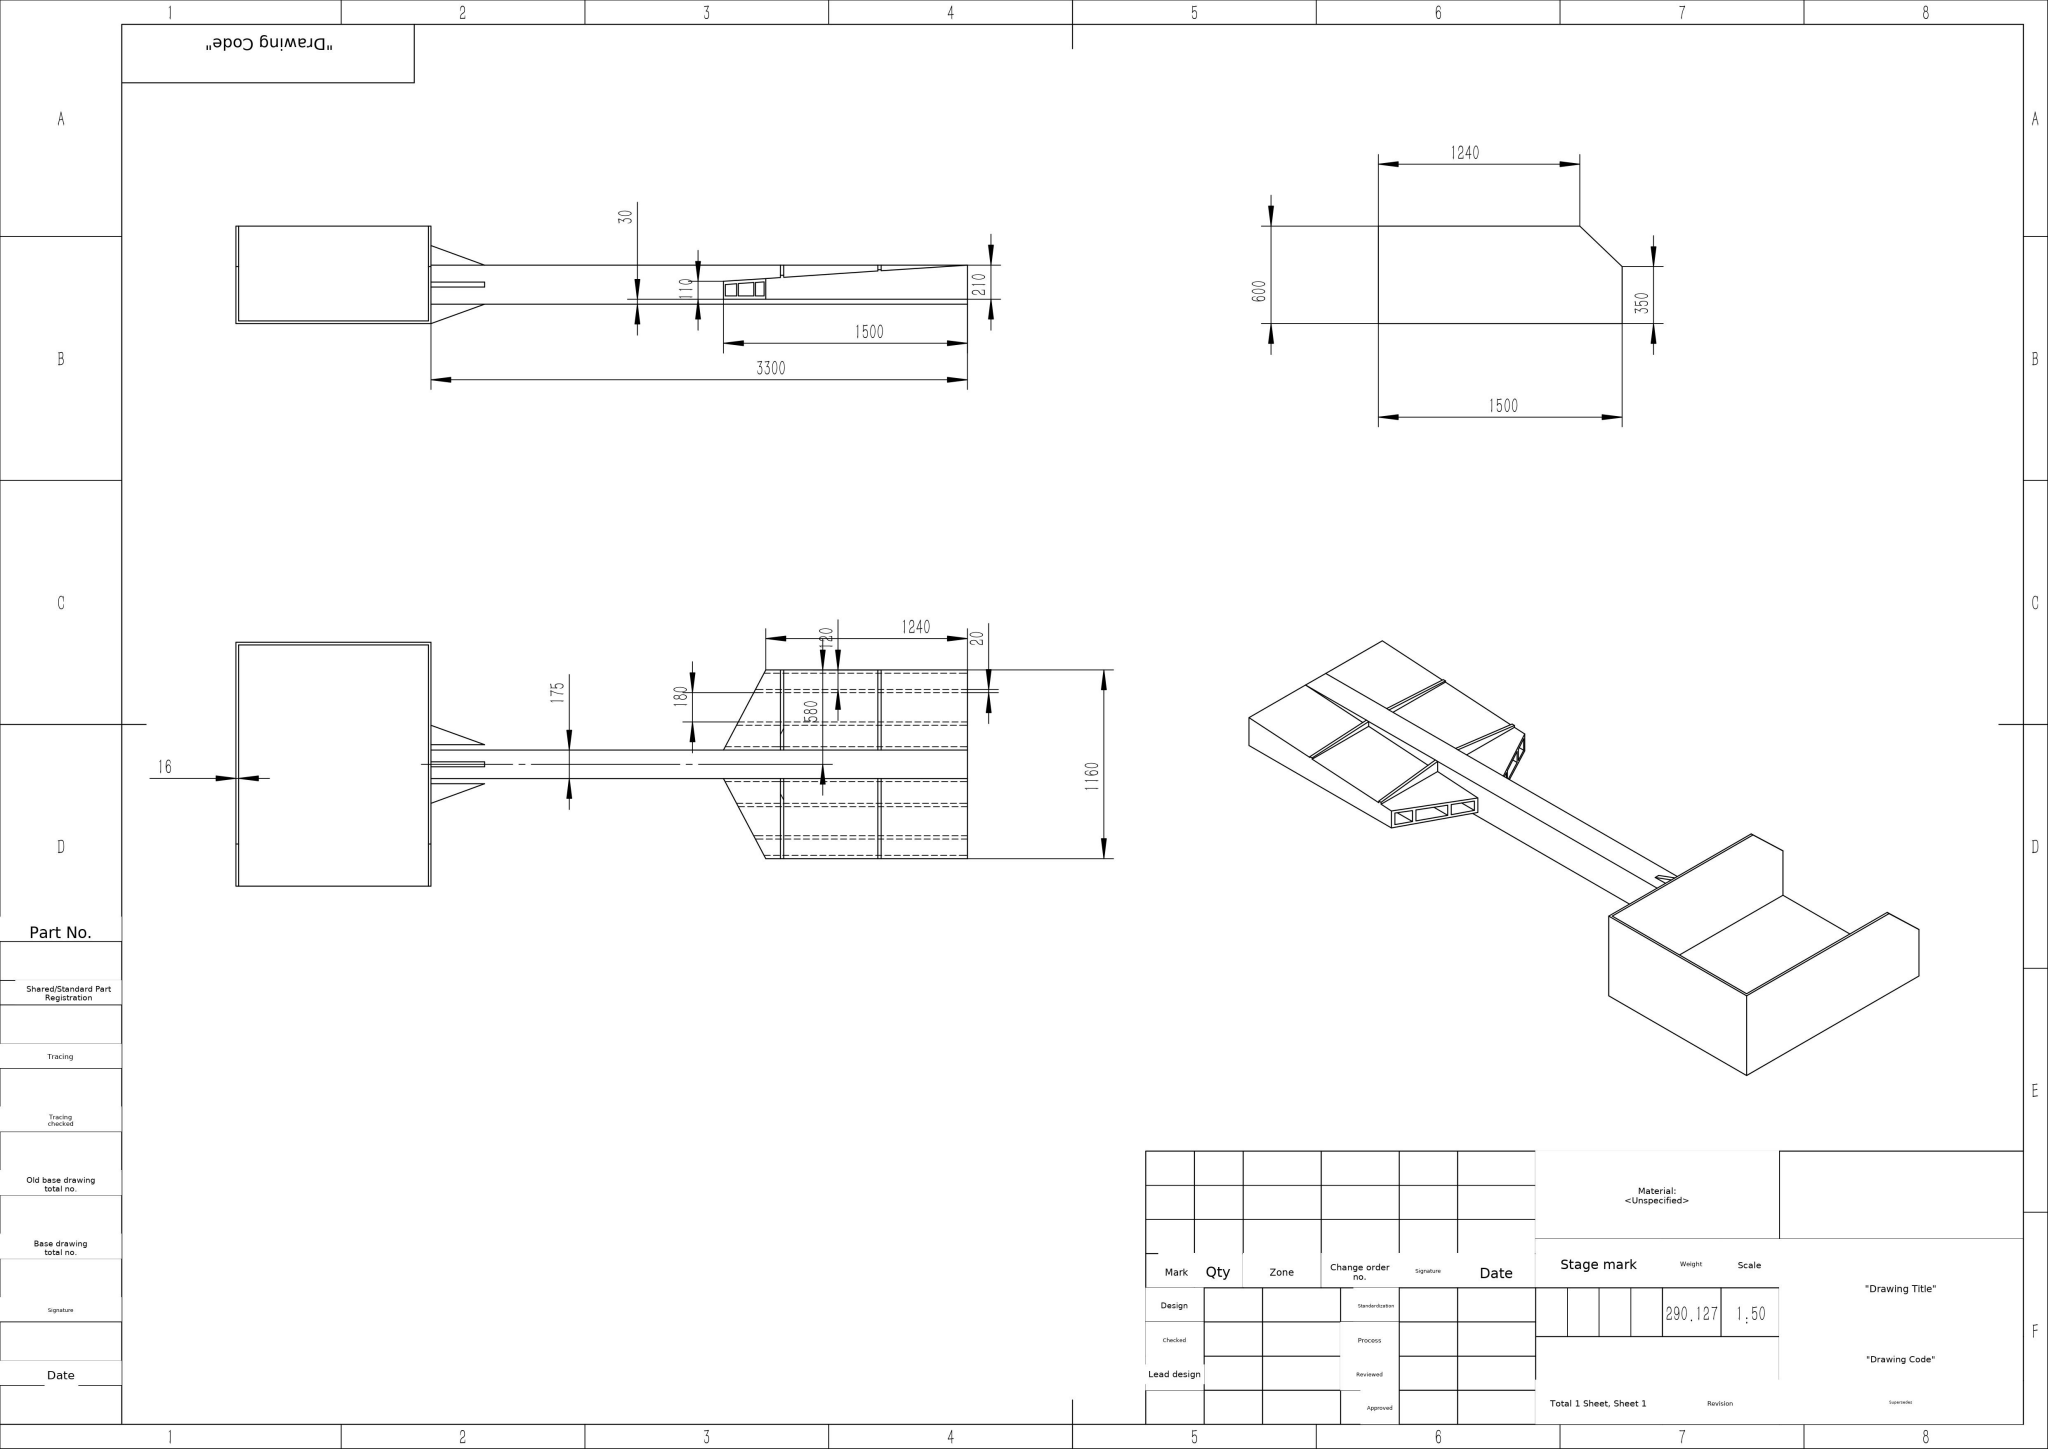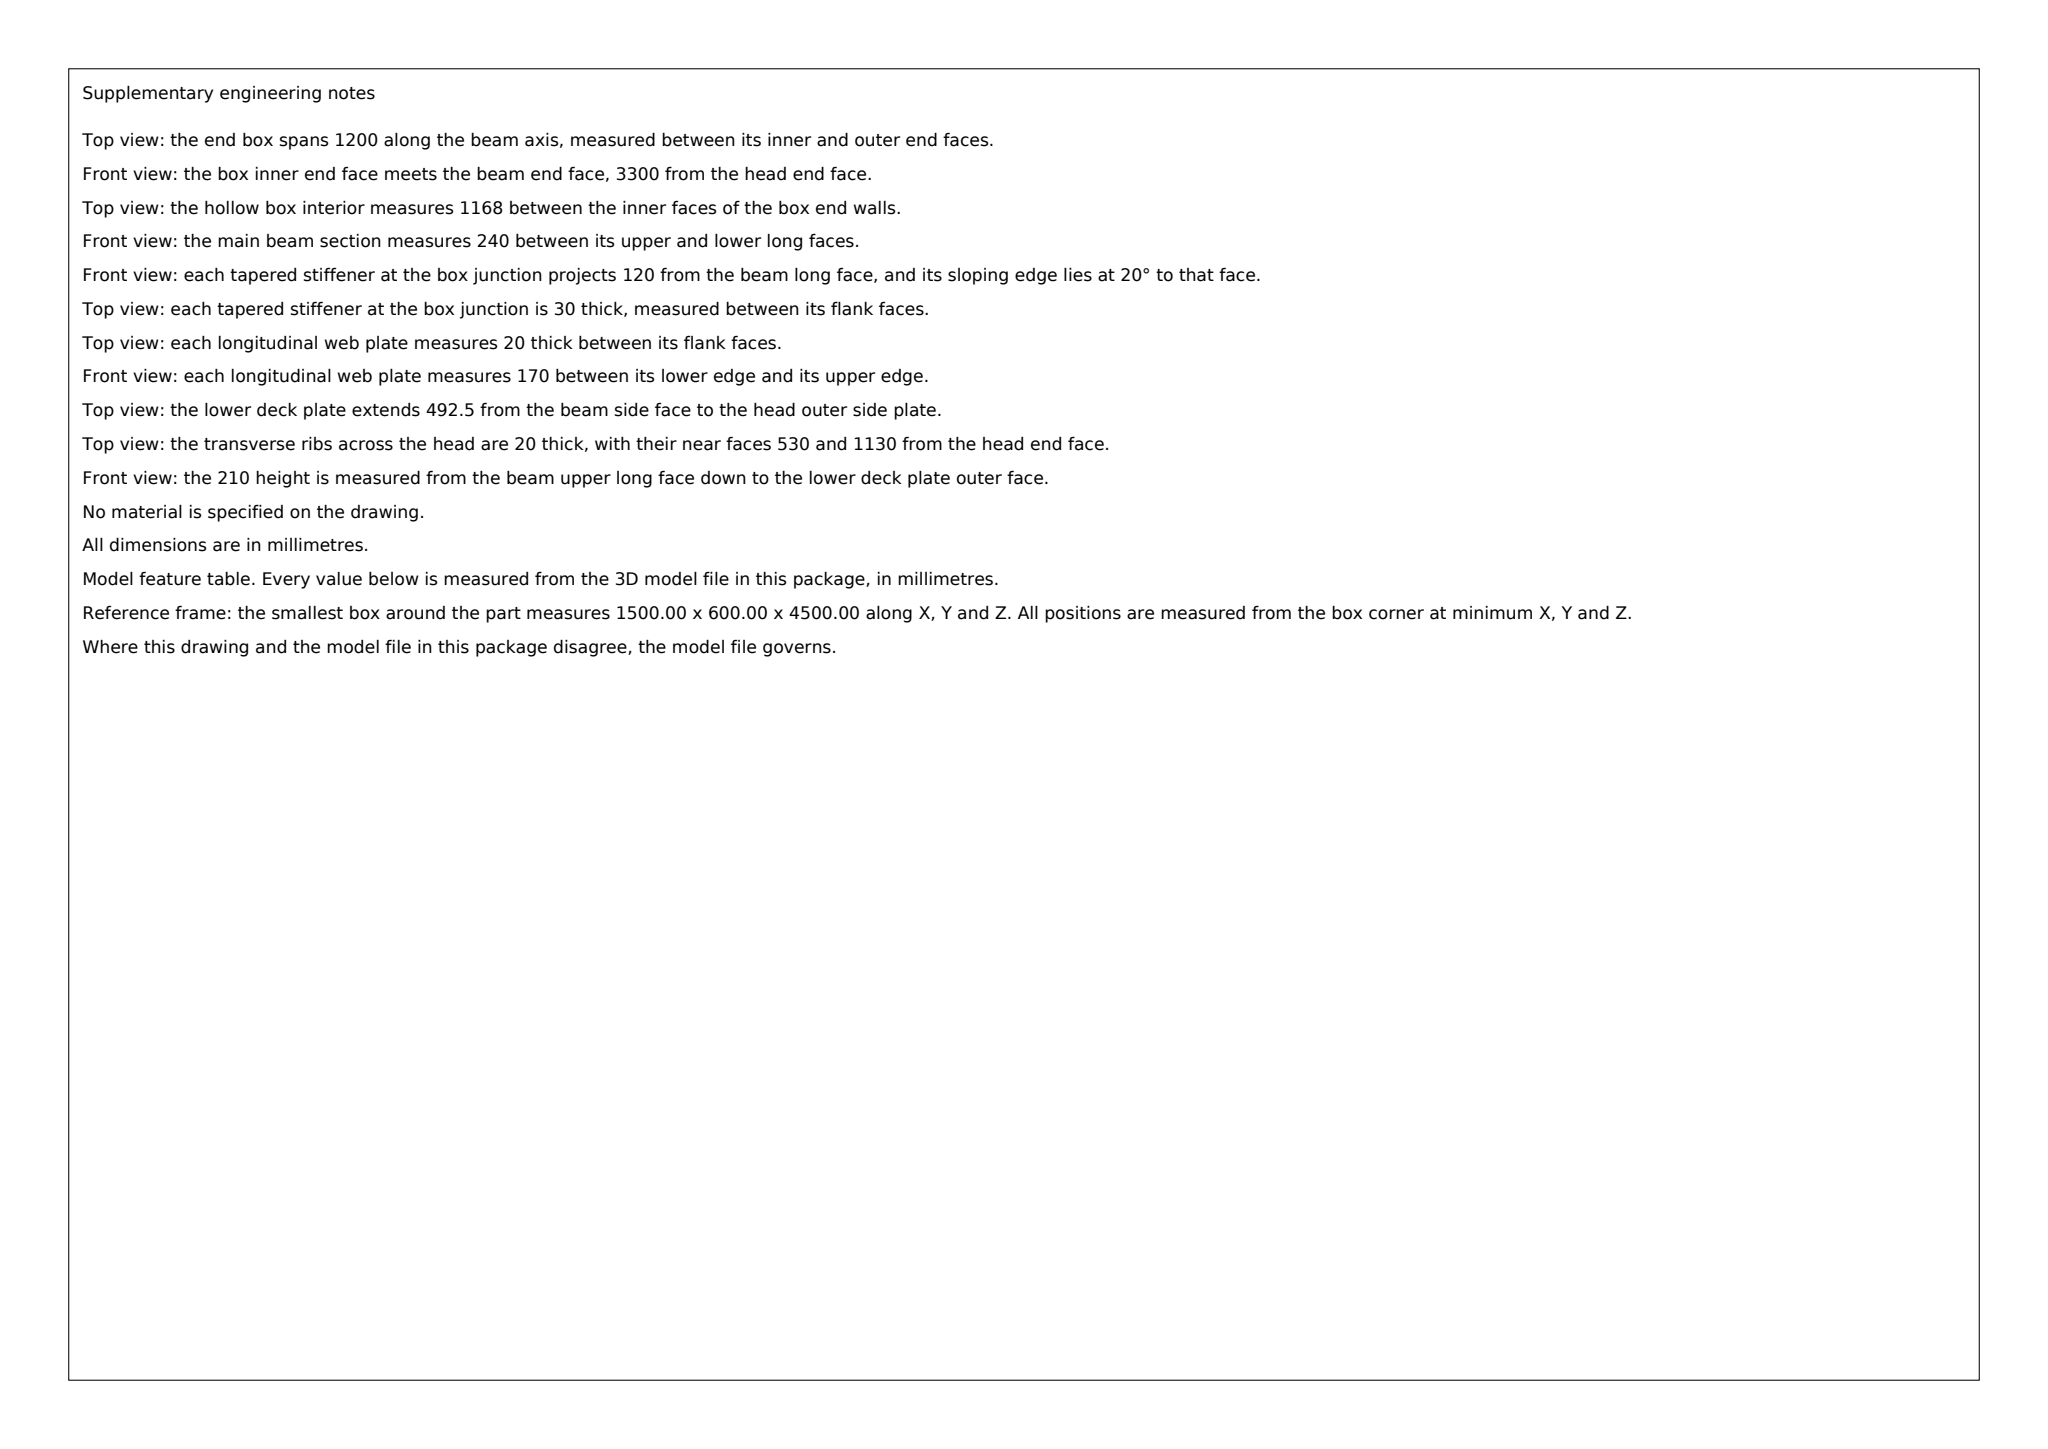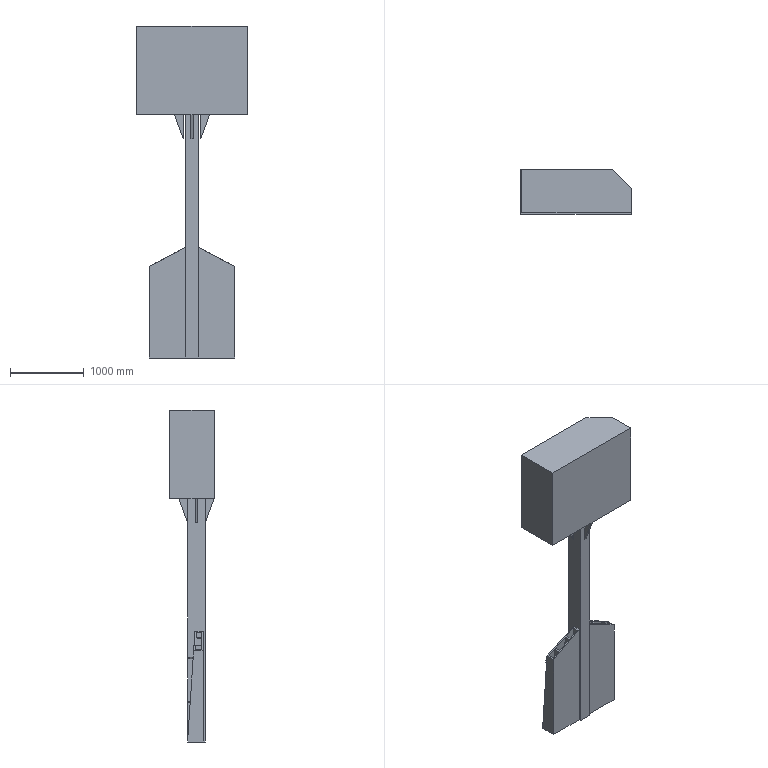Part | SolidWorks | mm | 1 solid | 89 faces | box 1500 x 600 x 4500 mm | volume 290127054 mm3 | plane 89
Drawing notes:
4X LONGL DECK PL 20 THK, CL AT 250 & 450 EA SIDE OF DECK CL | from the solid: x planes 290/310, 490/510, 990/1010, 1190/1210; bbox x=1500, CL x=750
DECK BUILD-UP FROM BTM FACE: Y=16,120,150,170,225,255,360 | from the solid: y planes 0,16,120,150,170,225,255,360,600
MAIN BEAM FLG PL 20 THK, FACES 87.5 & 107.5 FROM BEAM CL | from the solid: x planes 642.5/662.5 & 837.5/857.5; beam x=630-870, CL x=750
MAIN BEAM DEPTH 190, Y170 TO Y360 FROM BTM FACE | from the solid: y planes 170 and 360 bounding beam section
ALL BOX PL 16 THK TYP (FLOOR & END WALLS) | from the solid: z 3300-3316, z 4484-4500, y 0-16, x 0-16/1484-1500
20° RAMP TAPER BEGINS AT BOX END FACE, 3300 FROM RAMP TIP | from the solid: z plane 3300 = box start; bbox z=4500, box 1200 lg
ITEM 5 TAPER PLATES: 20°, START AT BOX FACE, 330 LG, 120 EA SIDE | from the solid: Box front wall plane z=3300 (beam 3300 LG to tip); beam side planes x=630/870 (240 wide); plate outer ends x=510/990 = 120 offset ea side; 120/tan20° = 330 plan length; 30 THK plates at y=120/150 & y=225/255
build123d program:
from build123d import *

# Parameters (mm, degrees)
SKETCH1_W               = 175
SKETCH1_H               = 240
BOSS_EXTRUDE1_DEPTH     = 3300
BOSS_EXTRUDE2_DEPTH     = 110
SKETCH4_W               = 1500
SKETCH4_H               = 600
BOSS_EXTRUDE3_DEPTH     = 1200
SKETCH5_W               = 1168
SKETCH5_H               = 1088.789
CUT_EXTRUDE2_DEPTH      = 1484
CUT_EXTRUDE3_DEPTH      = 3404.248
CUT_EXTRUDE3_DEPTH_BACK = 3404.248
BOSS_EXTRUDE4_DEPTH     = 15
CIRPATTERN1_COUNT       = 4
BOSS_EXTRUDE5_DEPTH     = 667.5
CUT_EXTRUDE4_DEPTH      = 30
BOSS_EXTRUDE6_REACH     = 4584.292
SKETCH18_W              = 20
SKETCH18_H              = 1436.319
SKETCH18_H_2            = 1605.271
CUT_EXTRUDE5_DEPTH      = 200
BOSS_EXTRUDE7_DEPTH     = 20
BOSS_EXTRUDE8_DEPTH     = 20


with BuildPart() as part:
    # Sketch1 → Boss-Extrude1 (new body)
    with BuildSketch(Plane.XY):
        Rectangle(SKETCH1_W, SKETCH1_H)
    extrude(amount=BOSS_EXTRUDE1_DEPTH)

    # Sketch2 → Boss-Extrude2 (add)
    with BuildSketch(Plane(origin=(0, -90, 0), x_dir=(-1, 0, 0), z_dir=(0, -1, 0))):
        Polygon((580, 0), (87.5, 0), (87.5, -1500), (580, -1240), align=None)
    boss_extrude2 = extrude(amount=-BOSS_EXTRUDE2_DEPTH)

    # Mirror1: Boss-Extrude2 across plane
    add(boss_extrude2.mirror(Plane(origin=(0, 0, 0), x_dir=(0, 0, 1), z_dir=(1, 0, 0))))

    # Sketch4 → Boss-Extrude3 (add)
    with BuildSketch(Plane.XY.offset(3300)):
        with Locations((0, 60)):
            Rectangle(SKETCH4_W, SKETCH4_H)
    extrude(amount=BOSS_EXTRUDE3_DEPTH)

    # Sketch5 → Cut-Extrude2 (cut)
    with BuildSketch(Plane(origin=(750, 0, 0), x_dir=(0, 0, -1), z_dir=(1, 0, 0))):
        with Locations((-3900, 320.394)):
            Rectangle(SKETCH5_W, SKETCH5_H)
    extrude(amount=-CUT_EXTRUDE2_DEPTH, mode=Mode.SUBTRACT)

    # Sketch6 → Cut-Extrude3 (cut, two sides: drawn at the far end of the back side and taken through both)
    with BuildSketch(Plane(origin=(0, 0, 3300), x_dir=(-1, 0, 0), z_dir=(0, 0, -1)).offset(-CUT_EXTRUDE3_DEPTH_BACK)):
        Polygon((-750, 110), (-490, 360), (-814.916, 501.7), align=None)
    extrude(amount=CUT_EXTRUDE3_DEPTH + CUT_EXTRUDE3_DEPTH_BACK, mode=Mode.SUBTRACT)

    # Sketch7 → Boss-Extrude4 (add, symmetric)
    with BuildSketch(Plane(origin=(0, 0, 0), x_dir=(0, 0, -1), z_dir=(1, 0, 0))):
        Polygon((-3300, 240), (-2970.303, 120), (-3300, 120), align=None)
    boss_extrude4 = extrude(amount=BOSS_EXTRUDE4_DEPTH, both=True)

    # CirPattern1: Boss-Extrude4 ×4 about axis
    cirpattern1_axis = Axis((0, 0, 0), (0, 0, 1))
    for i in range(1, CIRPATTERN1_COUNT):
        add(boss_extrude4.rotate(cirpattern1_axis, i * 360 / CIRPATTERN1_COUNT))

    # Sketch10 → Boss-Extrude5 (add)
    with BuildSketch(Plane(origin=(580, 0, 0), x_dir=(0, 0, -1), z_dir=(1, 0, 0))):
        Polygon((-1500, 20), (0, 120), (0, 20), align=None)
    boss_extrude5 = extrude(amount=-BOSS_EXTRUDE5_DEPTH)

    # Sketch12 → Cut-Extrude4 (cut)
    with BuildSketch(Plane.XZ.offset(-20)):
        Polygon((580, 1500), (87.5, 1500), (580, 1240), align=None)
    cut_extrude4 = extrude(amount=-CUT_EXTRUDE4_DEPTH, mode=Mode.SUBTRACT)

    # Mirror2: Boss-Extrude5, Cut-Extrude4 across plane
    add(boss_extrude5.mirror(Plane(origin=(0, 0, 0), x_dir=(0, 0, 1), z_dir=(1, 0, 0))))
    add(cut_extrude4.mirror(Plane(origin=(0, 0, 0), x_dir=(0, 0, 1), z_dir=(1, 0, 0))), mode=Mode.SUBTRACT)

    # Sketch17 → Cut-Loft1 section 0
    with BuildSketch(Plane(origin=(0, 0, 1500), x_dir=(-1, 0, 0), z_dir=(0, 0, -1))):
        with BuildLine():
            Line((-107.5, 0), (-560, 0))
            Line((-560, 0), (-560, -70))
            Line((-560, -70), (-107.5, -70))
            Line((-107.5, -70), (-107.5, 0))
        make_face()
    # Sketch14 → Cut-Loft1 section 1
    with BuildSketch(Plane(origin=(0, 0, 0), x_dir=(-1, 0, 0), z_dir=(0, 0, -1))):
        with BuildLine():
            Line((-560, 100), (-107.5, 100))
            Line((-107.5, 100), (-107.5, -70))
            Line((-107.5, -70), (-560, -70))
            Line((-560, -70), (-560, 100))
        make_face()
    cut_loft1 = loft(mode=Mode.SUBTRACT)

    # Boss-Extrude6: up to this plane
    boss_extrude6_end = Plane(origin=(0, 99.558, 6.637), z_dir=(0, -0.9978, -0.06652))
    # Sketch18 → Boss-Extrude6 (add, up to the surface)
    with BuildSketch(Plane(origin=(0, -70, 0), x_dir=(1, 0, 0), z_dir=(0, 1, 0)), mode=Mode.PRIVATE) as boss_extrude6_sk1:
        with Locations((450, -718.159)):
            Rectangle(SKETCH18_W, SKETCH18_H)
    boss_extrude6_tool1 = split(extrude(boss_extrude6_sk1.sketch, amount=BOSS_EXTRUDE6_REACH, mode=Mode.PRIVATE), bisect_by=boss_extrude6_end, keep=Keep.BOTH, mode=Mode.PRIVATE)
    # Sketch18 → Boss-Extrude6 (add, up to the surface)
    with BuildSketch(Plane(origin=(0, -70, 0), x_dir=(1, 0, 0), z_dir=(0, 1, 0)), mode=Mode.PRIVATE) as boss_extrude6_sk2:
        with Locations((250, -802.635)):
            Rectangle(SKETCH18_W, SKETCH18_H_2)
    boss_extrude6_tool2 = split(extrude(boss_extrude6_sk2.sketch, amount=BOSS_EXTRUDE6_REACH, mode=Mode.PRIVATE), bisect_by=boss_extrude6_end, keep=Keep.BOTH, mode=Mode.PRIVATE)
    boss_extrude6 = boss_extrude6_tool1.solids().sort_by_distance((450, -70, 718.159))[0] + boss_extrude6_tool2.solids().sort_by_distance((250, -70, 802.635))[0]
    add(boss_extrude6)

    # Sketch19 → Cut-Extrude5 (cut)
    with BuildSketch(Plane.XZ.offset(90)):
        Polygon((580, 1240), (87.5, 1500), (284.473, 1873.112), align=None)
    cut_extrude5 = extrude(amount=-CUT_EXTRUDE5_DEPTH, mode=Mode.SUBTRACT)

    # Mirror3: Cut-Loft1, Boss-Extrude6, Cut-Extrude5 across plane
    add(cut_loft1.mirror(Plane(origin=(0, 0, 0), x_dir=(0, 0, 1), z_dir=(1, 0, 0))), mode=Mode.SUBTRACT)
    add(boss_extrude6.mirror(Plane(origin=(0, 0, 0), x_dir=(0, 0, 1), z_dir=(1, 0, 0))))
    add(cut_extrude5.mirror(Plane(origin=(0, 0, 0), x_dir=(0, 0, 1), z_dir=(1, 0, 0))), mode=Mode.SUBTRACT)

    # Sketch21 → Boss-Extrude7 (add)
    with BuildSketch(Plane(origin=(0, 0, 1150), x_dir=(-1, 0, 0), z_dir=(0, 0, -1))):
        Polygon((-580, 37.333), (-87.5, 20), (-87.5, 120), (-580, 57.333), align=None)
    boss_extrude7 = extrude(amount=BOSS_EXTRUDE7_DEPTH)

    # Sketch24 → Boss-Extrude8 (add)
    with BuildSketch(Plane(origin=(0, 0, 550), x_dir=(-1, 0, 0), z_dir=(0, 0, -1))):
        Polygon((-87.5, 120), (-580, 91.912), (-580, 82.333), (-87.5, 82.333), align=None)
    boss_extrude8 = extrude(amount=BOSS_EXTRUDE8_DEPTH)

    # Mirror4: Boss-Extrude7, Boss-Extrude8 across plane
    add(boss_extrude7.mirror(Plane(origin=(0, 0, 0), x_dir=(0, 0, 1), z_dir=(1, 0, 0))))
    add(boss_extrude8.mirror(Plane(origin=(0, 0, 0), x_dir=(0, 0, 1), z_dir=(1, 0, 0))))


solid = part.part